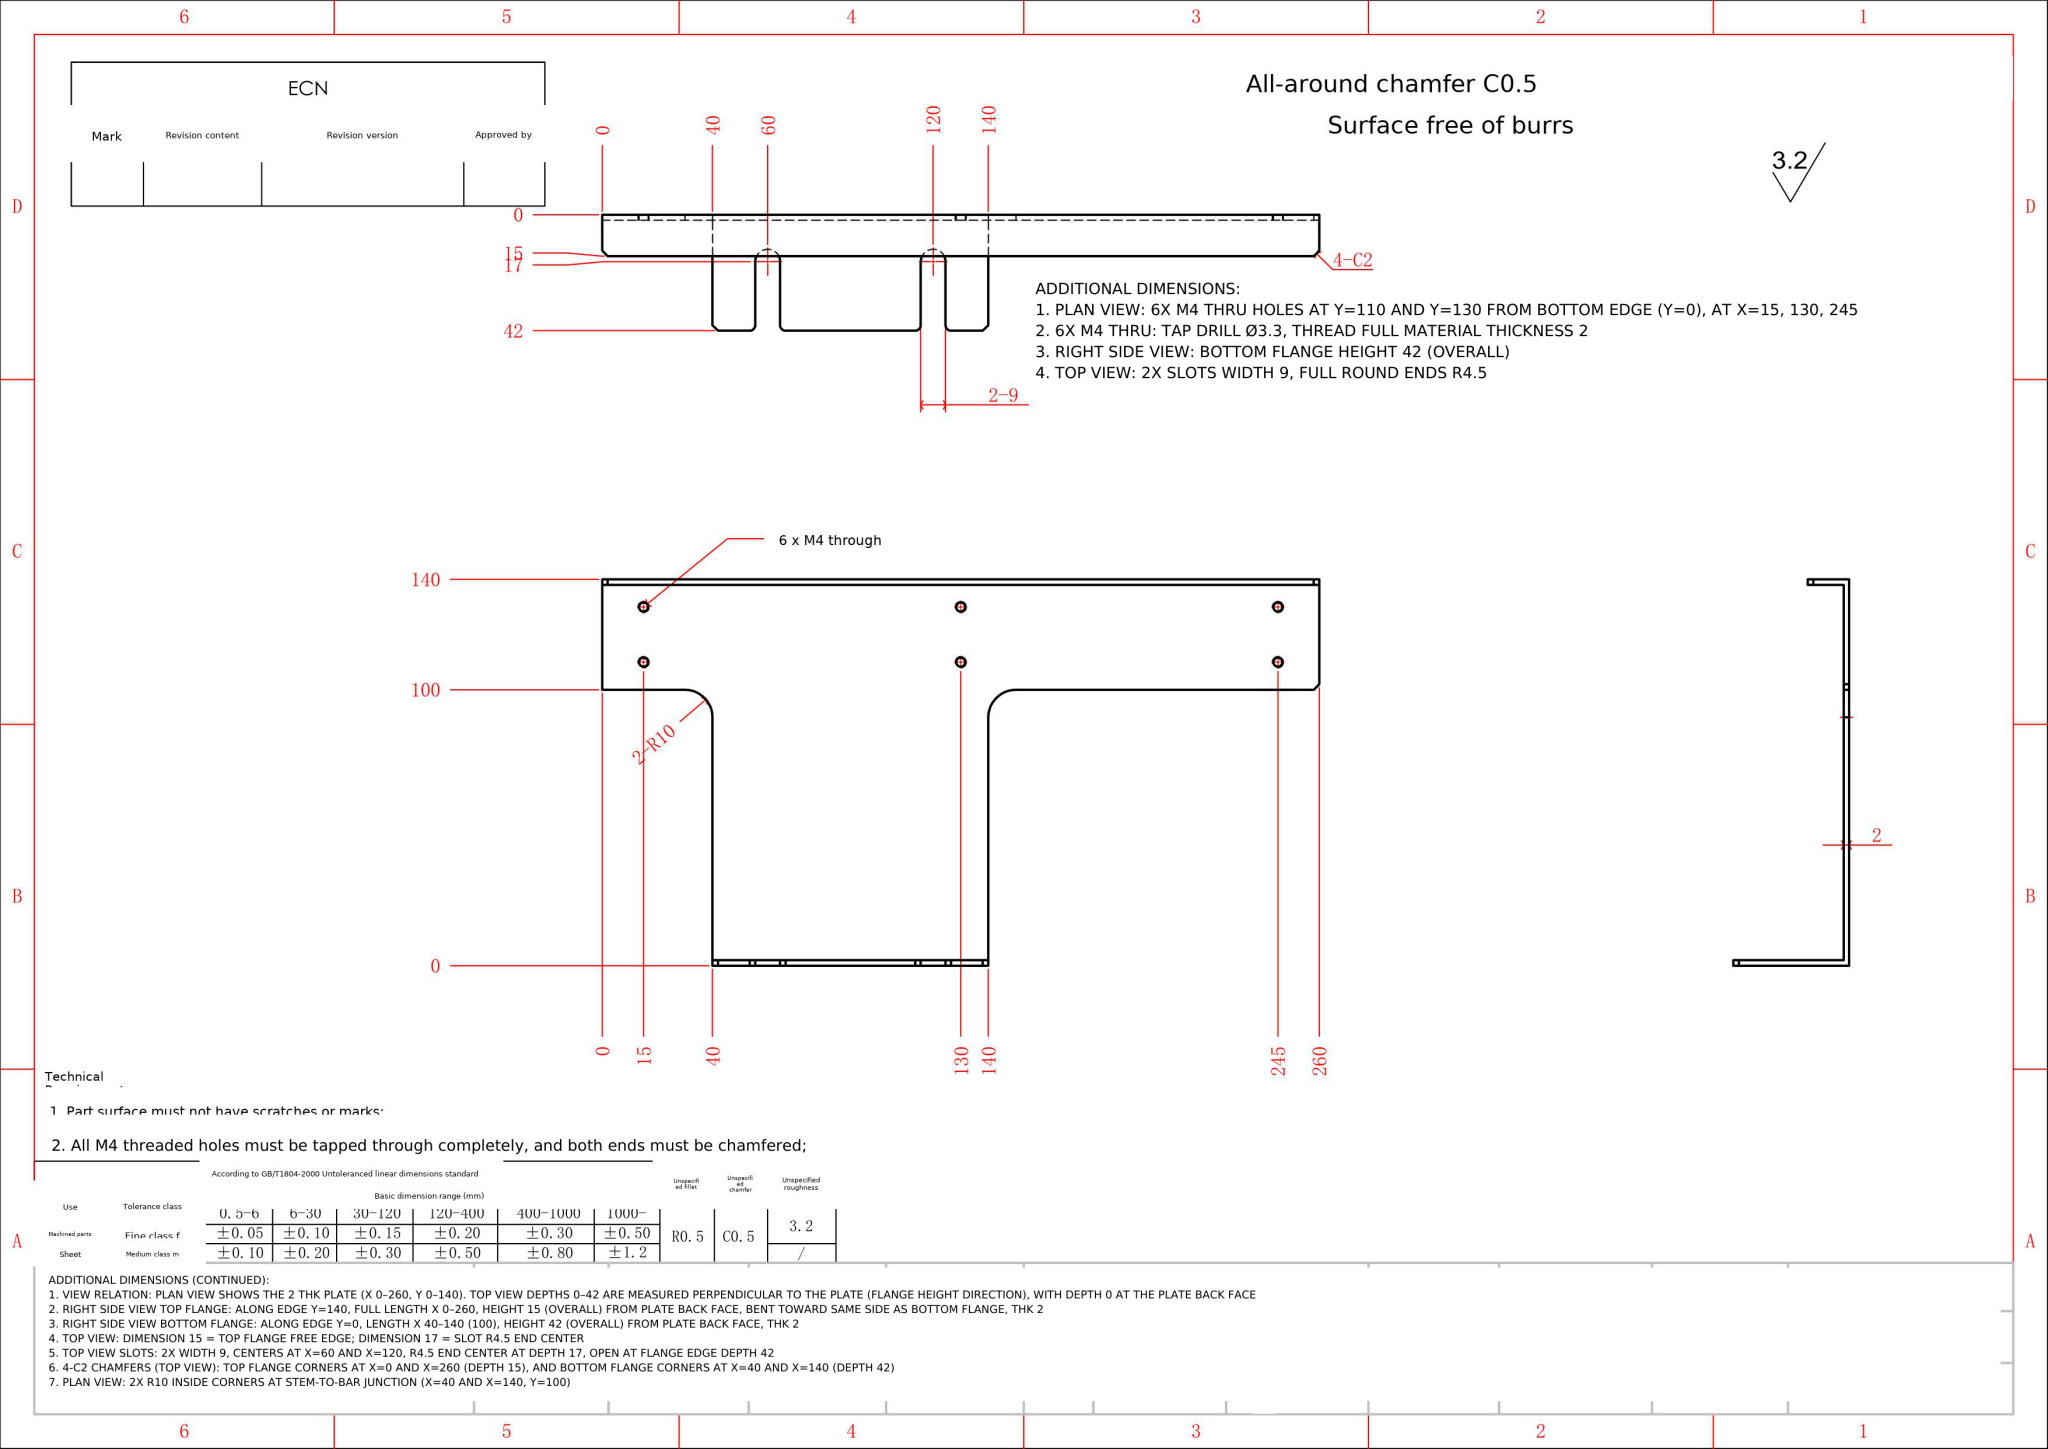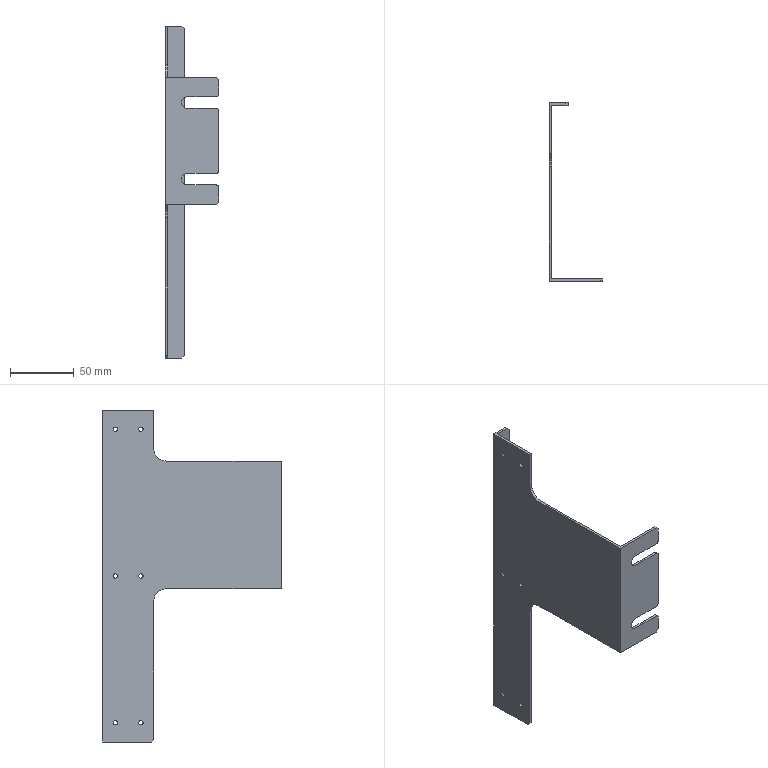Part | NX | mm | 1 solid | 45 faces | box 42 x 140 x 260 mm | volume 54489 mm3 | plane 25 | cylinder 20 | commonest cylinder face diameters 3.3 x12 4 x4 20 x2 9 x2